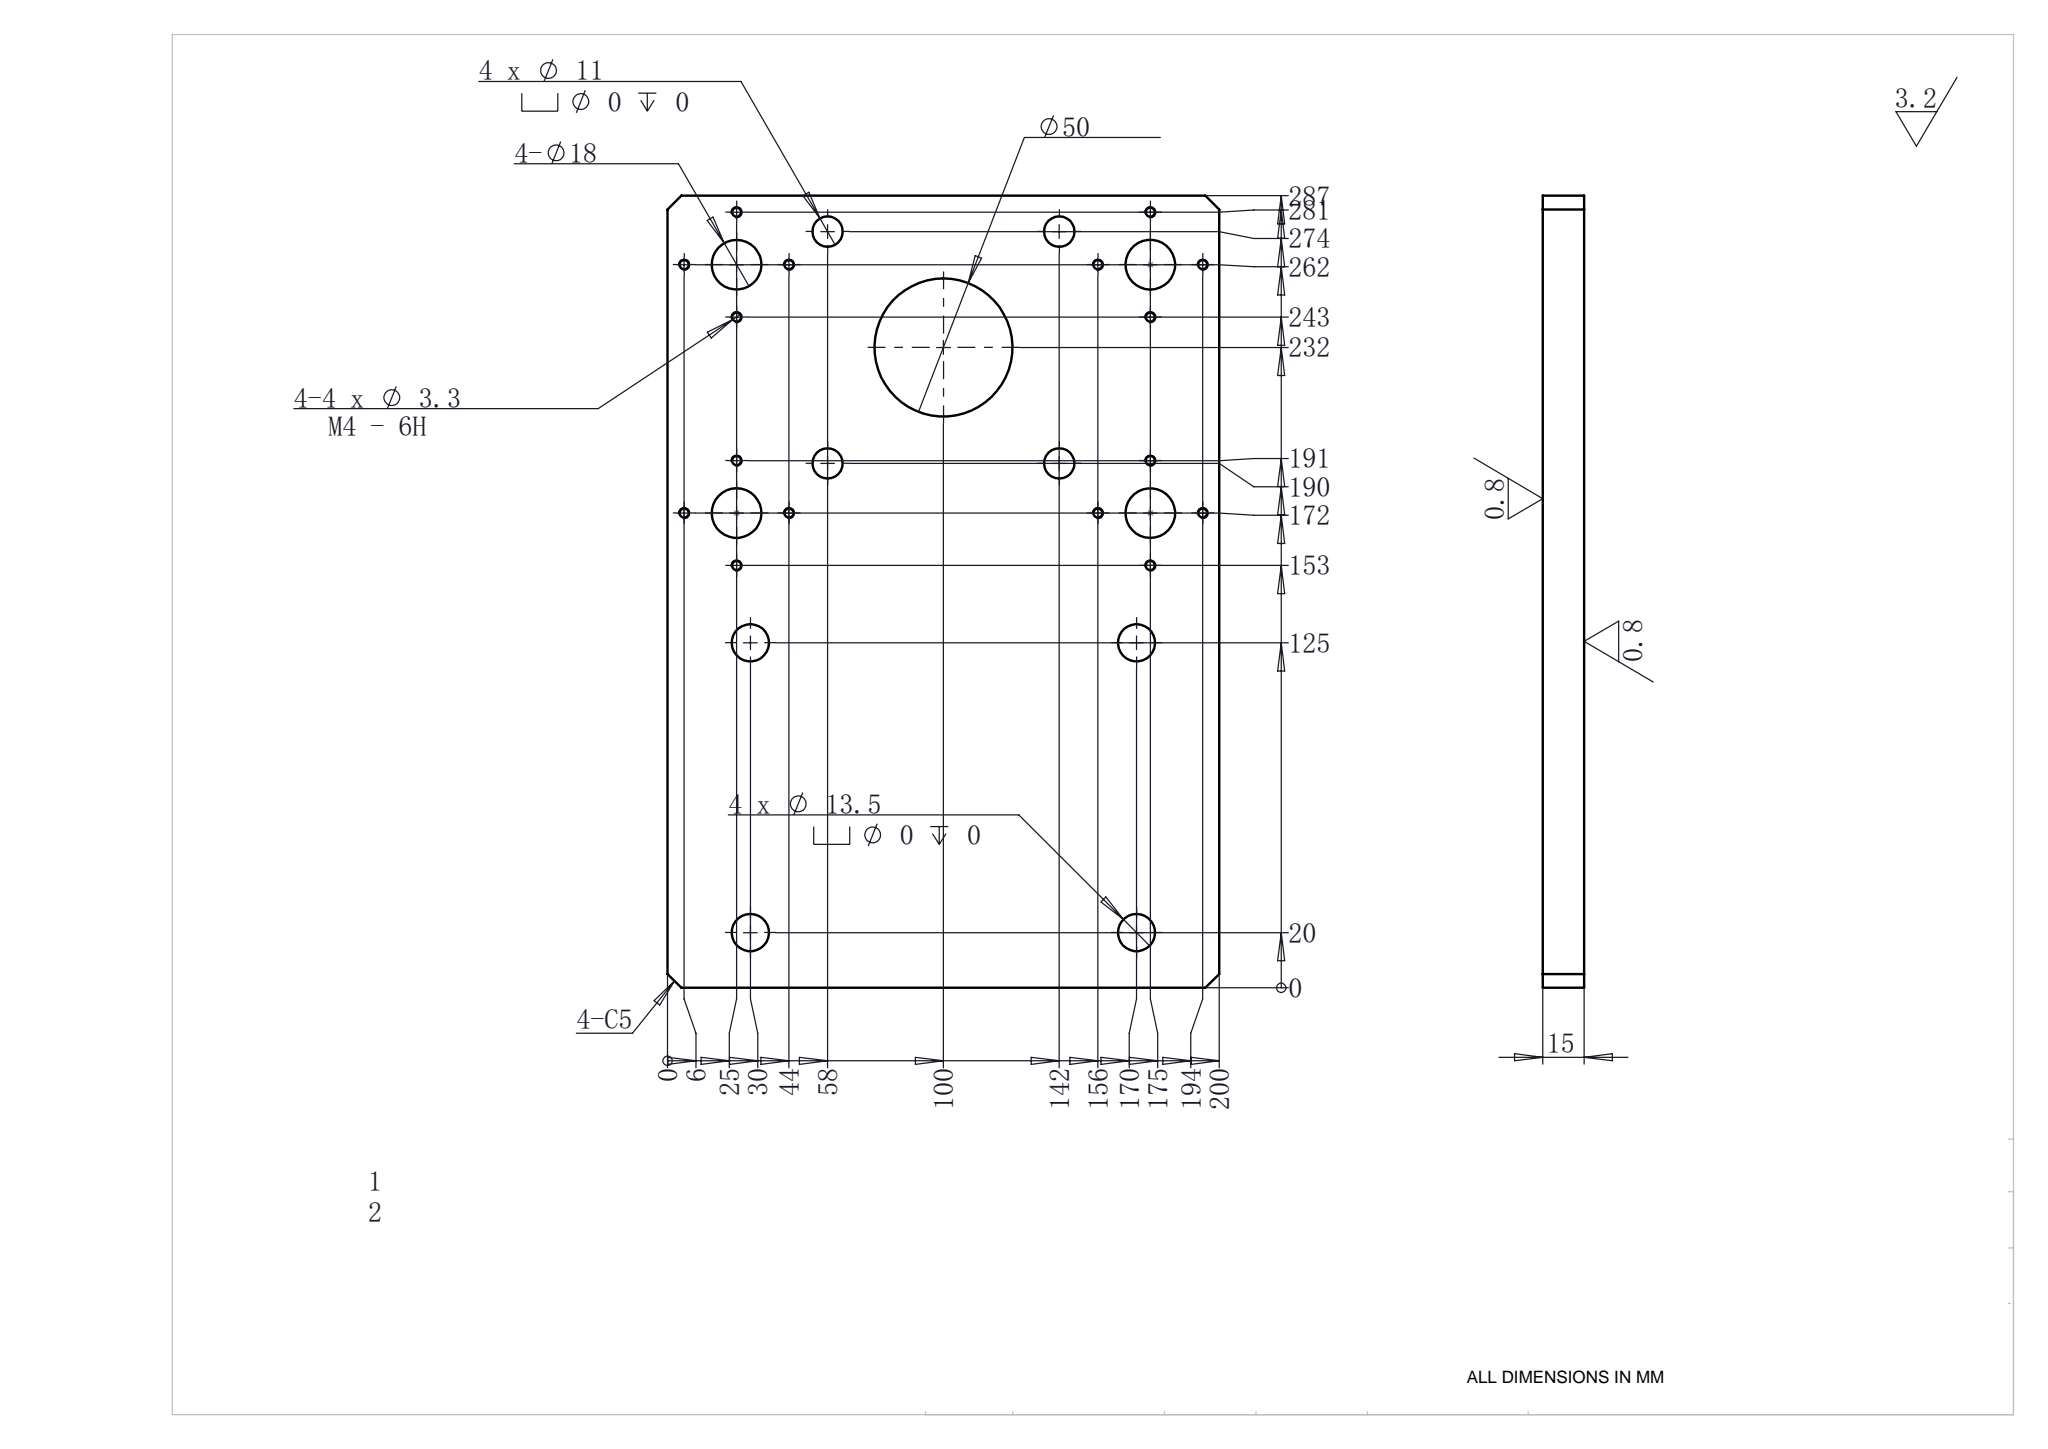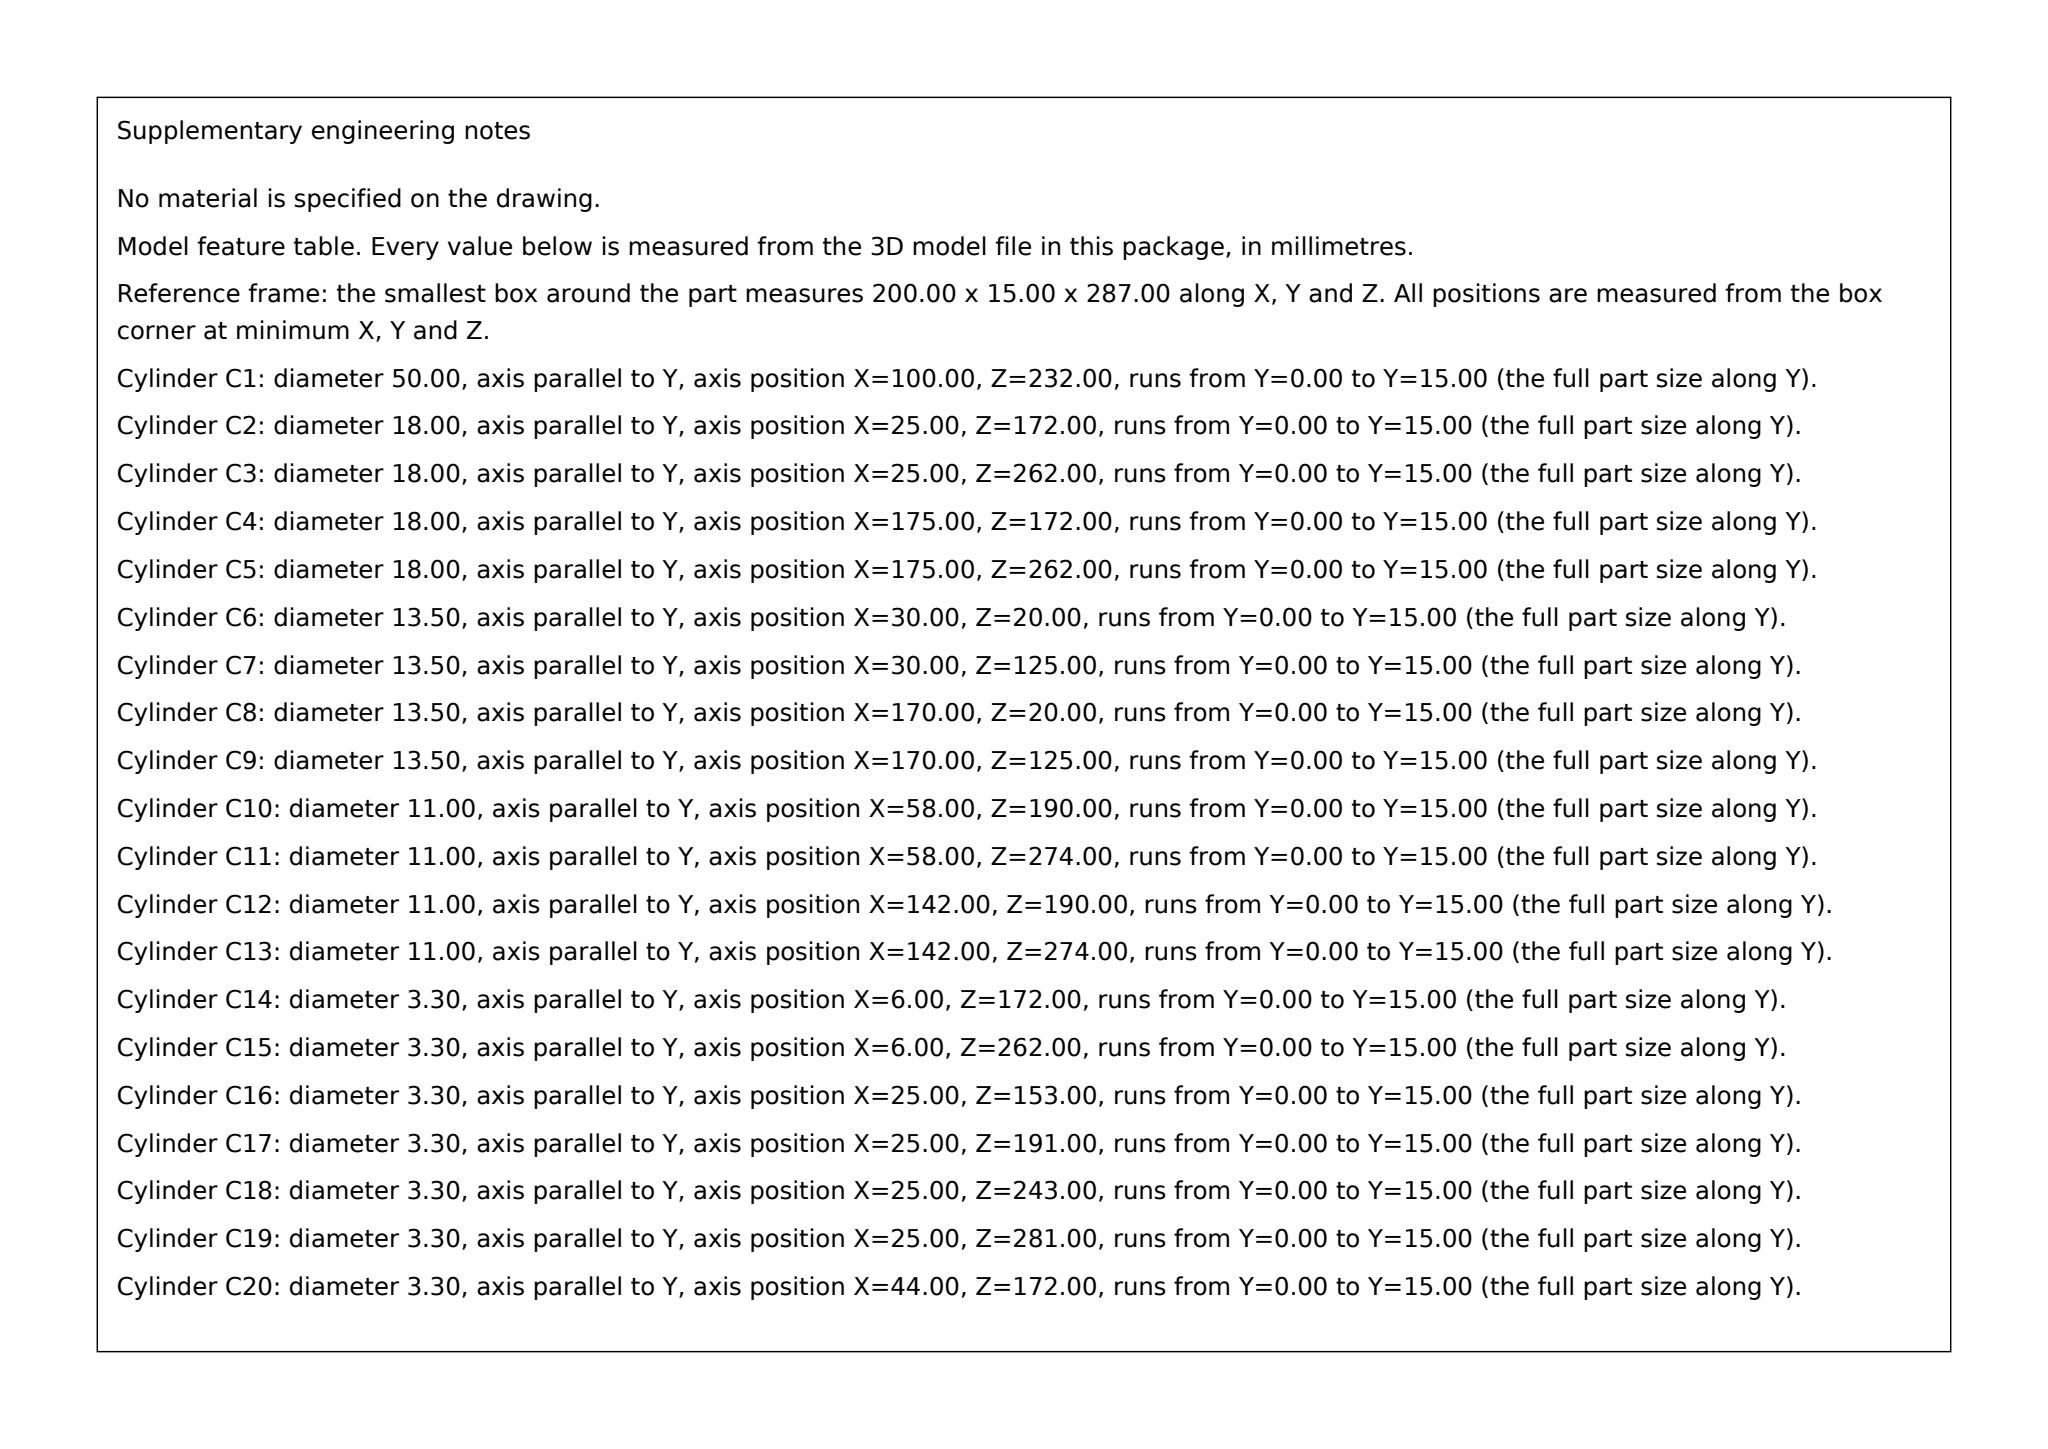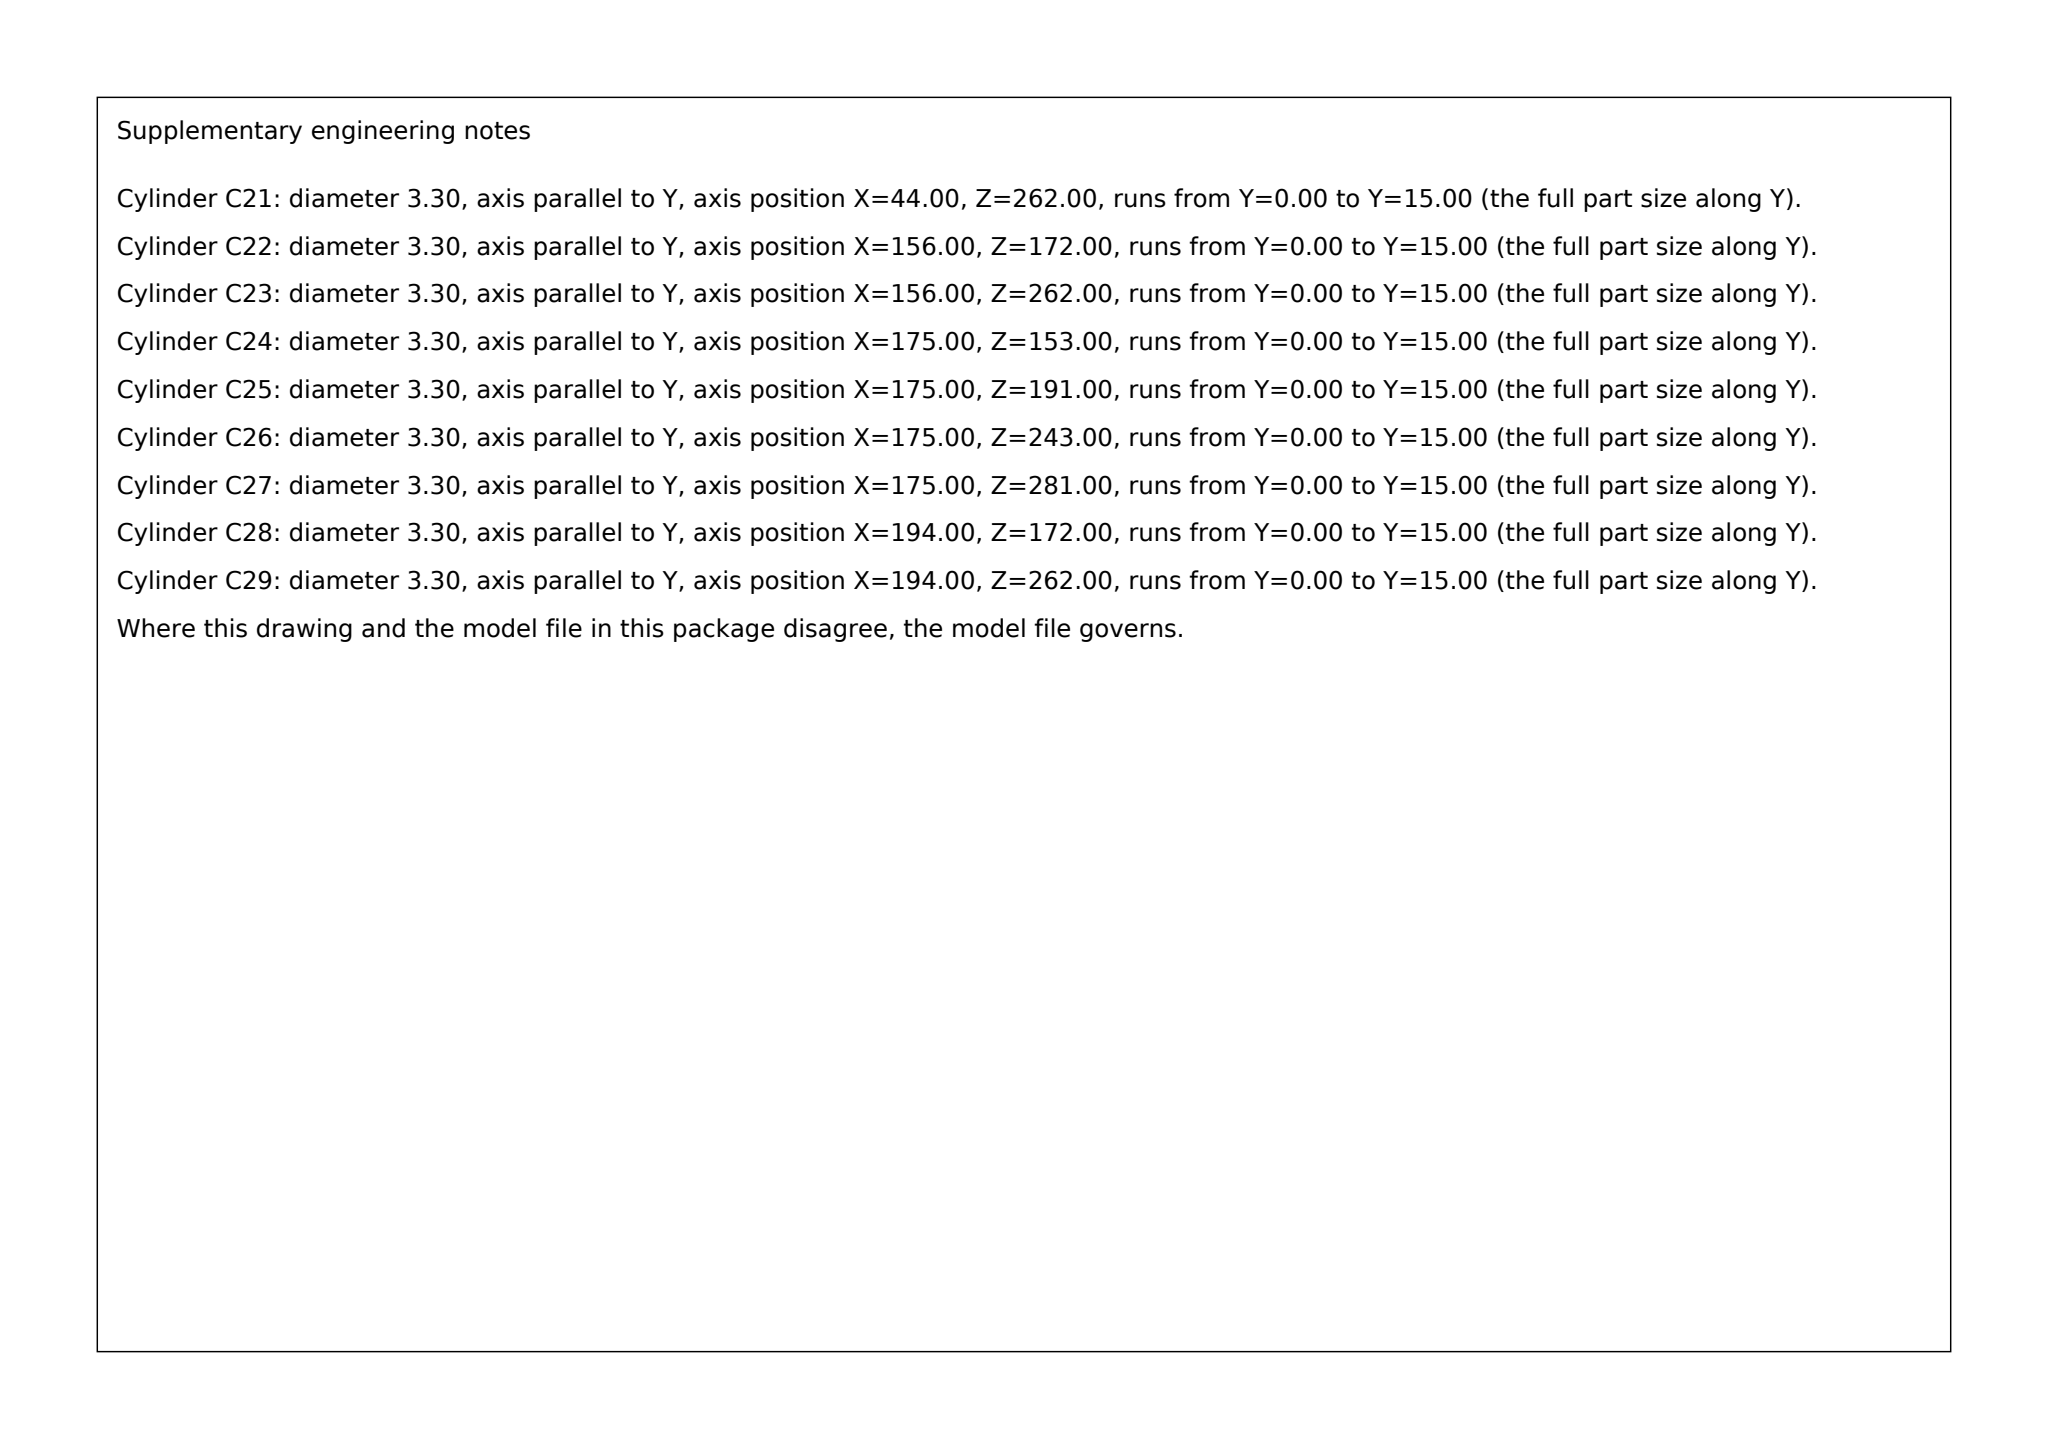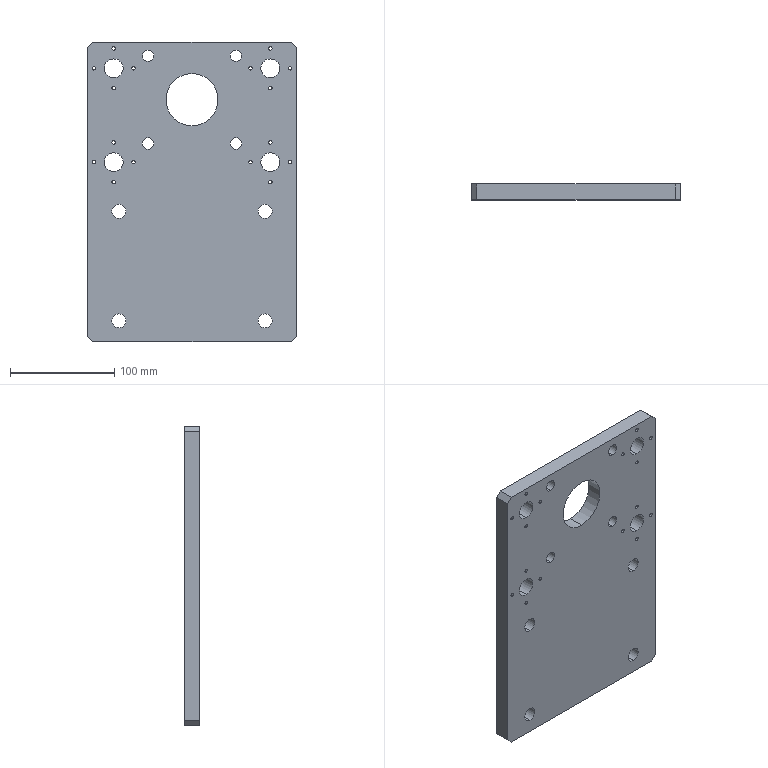Part | SolidWorks | mm | 1 solid | 68 faces | box 200 x 15 x 287 mm | volume 799186 mm3 | cylinder 58 | plane 10 | commonest cylinder face diameters 3.3 x32 13.5 x8 18 x8 11 x8 50 x2